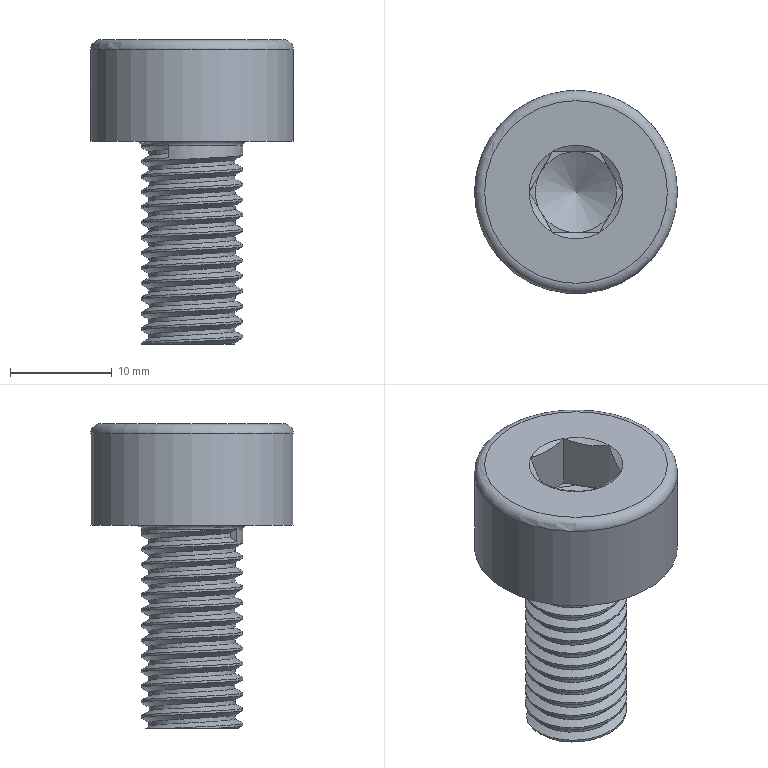Component | NX | M10X20_INT | 1 solid | 30 faces | volume 4011 mm3 | plane 16 | cone 7 | cylinder 3 | torus 2 | spline 2 | commonest cylinder face diameters 10 x1 20 x1 8.5 x1